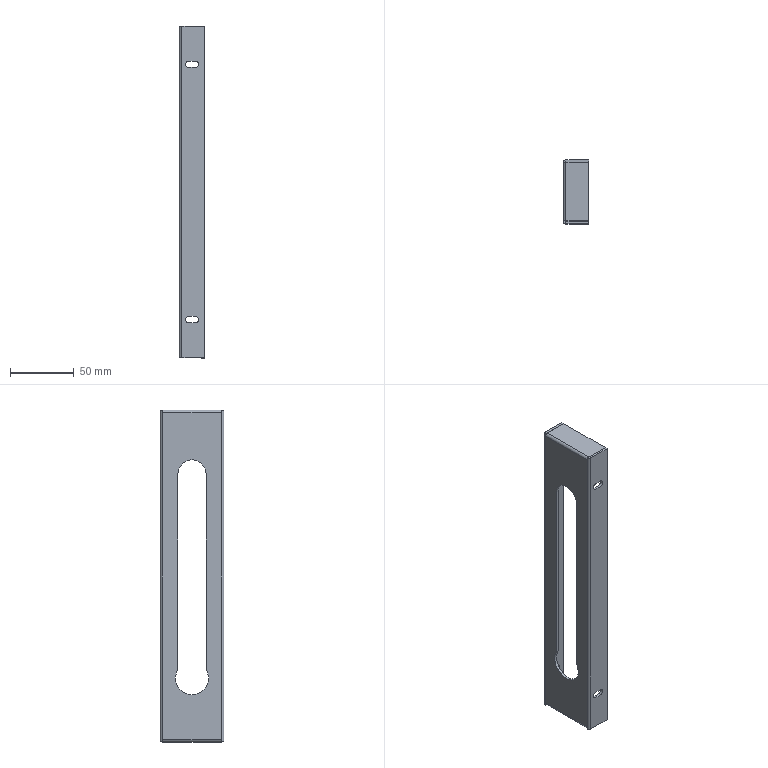Component | SolidWorks | GuideRail2-1 | 1 solid | 67 faces | volume 39094 mm3 | plane 44 | cylinder 23 | commonest cylinder face diameters 5 x12 4.2 x4 0.2 x4 22 x2 26 x1